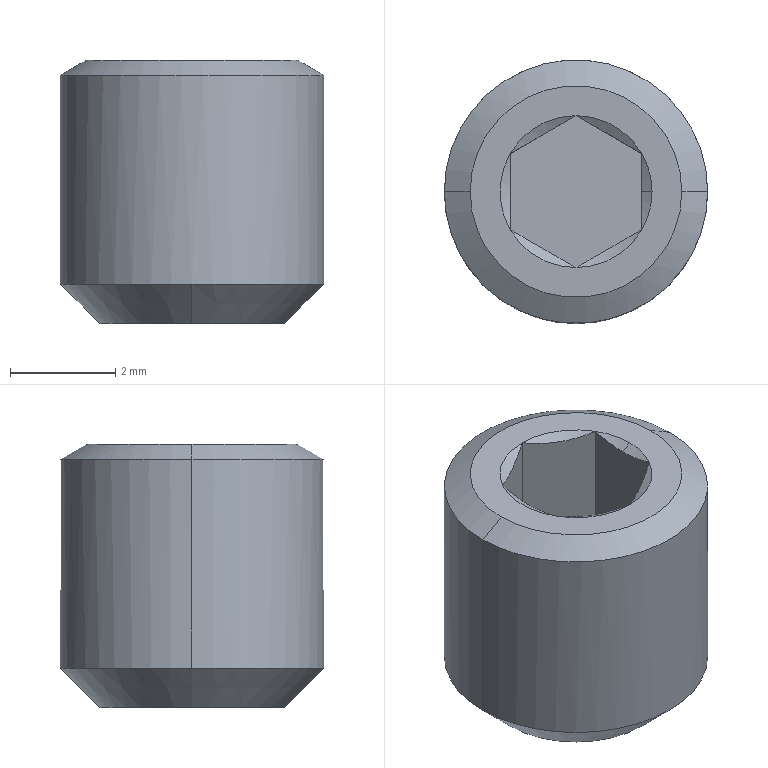Component | SolidWorks | DGC-18-280-G-PPV-A-1_HI_DIN-913 - M5x5_1-1 | 1 solid | 22 faces | box 5 x 5 x 5 mm | volume 82 mm3 | cone 11 | plane 9 | cylinder 2 | commonest cylinder face diameters 5 x2
STEP:
#1=COLOUR_RGB('',0.7922,0.8196,0.9333);
#2=FILL_AREA_STYLE_COLOUR('',#1);
#3=FILL_AREA_STYLE('',(#2));
#4=SURFACE_STYLE_FILL_AREA(#3);
#5=SURFACE_SIDE_STYLE('',(#4));
#6=SURFACE_STYLE_USAGE(.BOTH.,#5);
#7=PRESENTATION_STYLE_ASSIGNMENT((#6));
#8=CARTESIAN_POINT('',(2.476,17.604,4.802));
#9=VERTEX_POINT('',#8);
#10=CARTESIAN_POINT('',(2.673,17.604,4.802));
#11=VERTEX_POINT('',#10);
#12=CARTESIAN_POINT('',(2.575,17.604,4.802));
#13=DIRECTION('',(-0.,-0.,-1.));
#14=DIRECTION('',(-1.,0.,0.));
#15=AXIS2_PLACEMENT_3D('',#12,#13,#14);
#16=CIRCLE('',#15,0.09843);
#17=EDGE_CURVE('',#9,#11,#16,.T.);
#18=ORIENTED_EDGE('',*,*,#17,.T.);
#19=CARTESIAN_POINT('',(2.673,17.604,4.646));
#20=VERTEX_POINT('',#19);
#21=CARTESIAN_POINT('',(2.673,17.604,4.78));
#22=DIRECTION('',(-0.,-0.,-1.));
#23=VECTOR('',#22,39.37);
#24=LINE('',#21,#23);
#25=EDGE_CURVE('',#11,#20,#24,.T.);
#26=ORIENTED_EDGE('',*,*,#25,.T.);
#27=CARTESIAN_POINT('',(2.575,17.702,4.646));
#28=VERTEX_POINT('',#27);
#29=CARTESIAN_POINT('',(2.575,17.604,4.646));
#30=DIRECTION('',(0.,0.,1.));
#31=DIRECTION('',(-1.,0.,0.));
#32=AXIS2_PLACEMENT_3D('',#29,#30,#31);
#33=CIRCLE('',#32,0.09843);
#34=EDGE_CURVE('',#20,#28,#33,.T.);
#35=ORIENTED_EDGE('',*,*,#34,.T.);
#36=CARTESIAN_POINT('',(2.476,17.604,4.646));
#37=VERTEX_POINT('',#36);
#38=CARTESIAN_POINT('',(2.575,17.604,4.646));
#39=DIRECTION('',(0.,0.,1.));
#40=DIRECTION('',(-1.,0.,0.));
#41=AXIS2_PLACEMENT_3D('',#38,#39,#40);
#42=CIRCLE('',#41,0.09843);
#43=EDGE_CURVE('',#28,#37,#42,.T.);
#44=ORIENTED_EDGE('',*,*,#43,.T.);
#45=CARTESIAN_POINT('',(2.476,17.604,4.78));
#46=DIRECTION('',(-0.,-0.,-1.));
#47=VECTOR('',#46,39.37);
#48=LINE('',#45,#47);
#49=EDGE_CURVE('',#9,#37,#48,.T.);
#50=ORIENTED_EDGE('',*,*,#49,.F.);
#51=EDGE_LOOP('',(#18,#26,#35,#44,#50));
#52=FACE_OUTER_BOUND('',#51,.T.);
#53=CARTESIAN_POINT('',(2.575,17.604,4.78));
#54=DIRECTION('',(-0.,-0.,-1.));
#55=DIRECTION('',(-1.,0.,0.));
#56=AXIS2_PLACEMENT_3D('',#53,#54,#55);
#57=CYLINDRICAL_SURFACE('',#56,0.09843);
#58=ADVANCED_FACE('',(#52),#57,.T.);
#59=CARTESIAN_POINT('',(2.575,17.673,4.616));
#60=VERTEX_POINT('',#59);
#61=CARTESIAN_POINT('',(2.575,17.535,4.616));
#62=VERTEX_POINT('',#61);
#63=CARTESIAN_POINT('',(2.575,17.604,4.616));
#64=DIRECTION('',(0.,0.,1.));
#65=DIRECTION('',(0.,1.,0.));
#66=AXIS2_PLACEMENT_3D('',#63,#64,#65);
#67=CIRCLE('',#66,0.0689);
#68=EDGE_CURVE('',#60,#62,#67,.T.);
#69=ORIENTED_EDGE('',*,*,#68,.T.);
#70=CARTESIAN_POINT('',(2.575,17.505,4.646));
#71=VERTEX_POINT('',#70);
#72=CARTESIAN_POINT('',(2.575,17.505,4.646));
#73=DIRECTION('',(-0.,-0.7071,0.7071));
#74=VECTOR('',#73,39.37);
#75=LINE('',#72,#74);
#76=EDGE_CURVE('',#62,#71,#75,.T.);
#77=ORIENTED_EDGE('',*,*,#76,.T.);
#78=CARTESIAN_POINT('',(2.575,17.604,4.646));
#79=DIRECTION('',(0.,0.,1.));
#80=DIRECTION('',(-1.,0.,0.));
#81=AXIS2_PLACEMENT_3D('',#78,#79,#80);
#82=CIRCLE('',#81,0.09843);
#83=EDGE_CURVE('',#37,#71,#82,.T.);
#84=ORIENTED_EDGE('',*,*,#83,.F.);
#85=ORIENTED_EDGE('',*,*,#43,.F.);
#86=CARTESIAN_POINT('',(2.575,17.702,4.646));
#87=DIRECTION('',(0.,0.7071,0.7071));
#88=VECTOR('',#87,39.37);
#89=LINE('',#86,#88);
#90=EDGE_CURVE('',#60,#28,#89,.T.);
#91=ORIENTED_EDGE('',*,*,#90,.F.);
#92=EDGE_LOOP('',(#69,#77,#84,#85,#91));
#93=FACE_OUTER_BOUND('',#92,.T.);
#94=CARTESIAN_POINT('',(2.575,17.604,4.646));
#95=DIRECTION('',(0.,0.,1.));
#96=DIRECTION('',(0.,1.,0.));
#97=AXIS2_PLACEMENT_3D('',#94,#95,#96);
#98=CONICAL_SURFACE('',#97,0.09843,0.7854);
#99=ADVANCED_FACE('',(#93),#98,.T.);
#100=CARTESIAN_POINT('',(2.496,17.604,4.813));
#101=VERTEX_POINT('',#100);
#102=CARTESIAN_POINT('',(2.654,17.604,4.813));
#103=VERTEX_POINT('',#102);
#104=CARTESIAN_POINT('',(2.575,17.604,4.813));
#105=DIRECTION('',(-0.,-0.,-1.));
#106=DIRECTION('',(-1.,0.,0.));
#107=AXIS2_PLACEMENT_3D('',#104,#105,#106);
#108=CIRCLE('',#107,0.07911);
#109=EDGE_CURVE('',#101,#103,#108,.T.);
#110=ORIENTED_EDGE('',*,*,#109,.T.);
#111=CARTESIAN_POINT('',(2.673,17.604,4.802));
#112=DIRECTION('',(0.866,0.,-0.5));
#113=VECTOR('',#112,39.37);
#114=LINE('',#111,#113);
#115=EDGE_CURVE('',#103,#11,#114,.T.);
#116=ORIENTED_EDGE('',*,*,#115,.T.);
#117=ORIENTED_EDGE('',*,*,#17,.F.);
#118=CARTESIAN_POINT('',(2.476,17.604,4.802));
#119=DIRECTION('',(-0.866,-0.,-0.5));
#120=VECTOR('',#119,39.37);
#121=LINE('',#118,#120);
#122=EDGE_CURVE('',#101,#9,#121,.T.);
#123=ORIENTED_EDGE('',*,*,#122,.F.);
#124=EDGE_LOOP('',(#110,#116,#117,#123));
#125=FACE_OUTER_BOUND('',#124,.T.);
#126=CARTESIAN_POINT('',(2.575,17.604,4.802));
#127=DIRECTION('',(-0.,-0.,-1.));
#128=DIRECTION('',(-1.,0.,0.));
#129=AXIS2_PLACEMENT_3D('',#126,#127,#128);
#130=CONICAL_SURFACE('',#129,0.09843,1.047);
#131=ADVANCED_FACE('',(#125),#130,.T.);
#132=CARTESIAN_POINT('',(2.624,17.604,4.809));
#133=VERTEX_POINT('',#132);
#134=CARTESIAN_POINT('',(2.624,17.632,4.813));
#135=VERTEX_POINT('',#134);
#136=CARTESIAN_POINT('',(2.624,17.604,4.809));
#137=CARTESIAN_POINT('',(2.624,17.613,4.809));
#138=CARTESIAN_POINT('',(2.624,17.623,4.81));
#139=CARTESIAN_POINT('',(2.624,17.632,4.813));
#140=B_SPLINE_CURVE_WITH_KNOTS('',3,(#136,#137,#138,#139),.UNSPECIFIED.,.F.,.F.,(4,4),(0.0007302,0.001458),.UNSPECIFIED.);
#141=EDGE_CURVE('',#133,#135,#140,.T.);
#142=ORIENTED_EDGE('',*,*,#141,.F.);
#143=CARTESIAN_POINT('',(2.632,17.604,4.813));
#144=VERTEX_POINT('',#143);
#145=CARTESIAN_POINT('',(2.632,17.604,4.813));
#146=DIRECTION('',(0.866,0.,0.5));
#147=VECTOR('',#146,39.37);
#148=LINE('',#145,#147);
#149=EDGE_CURVE('',#133,#144,#148,.T.);
#150=ORIENTED_EDGE('',*,*,#149,.T.);
#151=CARTESIAN_POINT('',(2.575,17.604,4.813));
#152=DIRECTION('',(0.,0.,1.));
#153=DIRECTION('',(1.,0.,0.));
#154=AXIS2_PLACEMENT_3D('',#151,#152,#153);
#155=CIRCLE('',#154,0.05683);
#156=EDGE_CURVE('',#144,#135,#155,.T.);
#157=ORIENTED_EDGE('',*,*,#156,.T.);
#158=EDGE_LOOP('',(#142,#150,#157));
#159=FACE_OUTER_BOUND('',#158,.T.);
#160=CARTESIAN_POINT('',(2.575,17.604,4.813));
#161=DIRECTION('',(0.,0.,1.));
#162=DIRECTION('',(1.,0.,0.));
#163=AXIS2_PLACEMENT_3D('',#160,#161,#162);
#164=CONICAL_SURFACE('',#163,0.05683,1.047);
#165=ADVANCED_FACE('',(#159),#164,.F.);
#166=ORIENTED_EDGE('',*,*,#25,.F.);
#167=CARTESIAN_POINT('',(2.575,17.604,4.802));
#168=DIRECTION('',(-0.,-0.,-1.));
#169=DIRECTION('',(-1.,0.,0.));
#170=AXIS2_PLACEMENT_3D('',#167,#168,#169);
#171=CIRCLE('',#170,0.09843);
#172=EDGE_CURVE('',#11,#9,#171,.T.);
#173=ORIENTED_EDGE('',*,*,#172,.T.);
#174=ORIENTED_EDGE('',*,*,#49,.T.);
#175=ORIENTED_EDGE('',*,*,#83,.T.);
#176=CARTESIAN_POINT('',(2.575,17.604,4.646));
#177=DIRECTION('',(0.,0.,1.));
#178=DIRECTION('',(-1.,0.,0.));
#179=AXIS2_PLACEMENT_3D('',#176,#177,#178);
#180=CIRCLE('',#179,0.09843);
#181=EDGE_CURVE('',#71,#20,#180,.T.);
#182=ORIENTED_EDGE('',*,*,#181,.T.);
#183=EDGE_LOOP('',(#166,#173,#174,#175,#182));
#184=FACE_OUTER_BOUND('',#183,.T.);
#185=CARTESIAN_POINT('',(2.575,17.604,4.78));
#186=DIRECTION('',(-0.,-0.,-1.));
#187=DIRECTION('',(-1.,0.,0.));
#188=AXIS2_PLACEMENT_3D('',#185,#186,#187);
#189=CYLINDRICAL_SURFACE('',#188,0.09843);
#190=ADVANCED_FACE('',(#184),#189,.T.);
#191=ORIENTED_EDGE('',*,*,#76,.F.);
#192=CARTESIAN_POINT('',(2.575,17.604,4.616));
#193=DIRECTION('',(0.,0.,1.));
#194=DIRECTION('',(0.,1.,0.));
#195=AXIS2_PLACEMENT_3D('',#192,#193,#194);
#196=CIRCLE('',#195,0.0689);
#197=EDGE_CURVE('',#62,#60,#196,.T.);
#198=ORIENTED_EDGE('',*,*,#197,.T.);
#199=ORIENTED_EDGE('',*,*,#90,.T.);
#200=ORIENTED_EDGE('',*,*,#34,.F.);
#201=ORIENTED_EDGE('',*,*,#181,.F.);
#202=EDGE_LOOP('',(#191,#198,#199,#200,#201));
#203=FACE_OUTER_BOUND('',#202,.T.);
#204=CARTESIAN_POINT('',(2.575,17.604,4.646));
#205=DIRECTION('',(0.,0.,1.));
#206=DIRECTION('',(0.,1.,0.));
#207=AXIS2_PLACEMENT_3D('',#204,#205,#206);
#208=CONICAL_SURFACE('',#207,0.09843,0.7854);
#209=ADVANCED_FACE('',(#203),#208,.T.);
#210=ORIENTED_EDGE('',*,*,#115,.F.);
#211=CARTESIAN_POINT('',(2.575,17.604,4.813));
#212=DIRECTION('',(-0.,-0.,-1.));
#213=DIRECTION('',(-1.,0.,0.));
#214=AXIS2_PLACEMENT_3D('',#211,#212,#213);
#215=CIRCLE('',#214,0.07911);
#216=EDGE_CURVE('',#103,#101,#215,.T.);
#217=ORIENTED_EDGE('',*,*,#216,.T.);
#218=ORIENTED_EDGE('',*,*,#122,.T.);
#219=ORIENTED_EDGE('',*,*,#172,.F.);
#220=EDGE_LOOP('',(#210,#217,#218,#219));
#221=FACE_OUTER_BOUND('',#220,.T.);
#222=CARTESIAN_POINT('',(2.575,17.604,4.802));
#223=DIRECTION('',(-0.,-0.,-1.));
#224=DIRECTION('',(-1.,0.,0.));
#225=AXIS2_PLACEMENT_3D('',#222,#223,#224);
#226=CONICAL_SURFACE('',#225,0.09843,1.047);
#227=ADVANCED_FACE('',(#221),#226,.T.);
#228=ORIENTED_EDGE('',*,*,#68,.F.);
#229=ORIENTED_EDGE('',*,*,#197,.F.);
#230=EDGE_LOOP('',(#228,#229));
#231=FACE_OUTER_BOUND('',#230,.T.);
#232=CARTESIAN_POINT('',(2.575,17.604,4.616));
#233=DIRECTION('',(0.,0.,1.));
#234=DIRECTION('',(1.,0.,-0.));
#235=AXIS2_PLACEMENT_3D('',#232,#233,#234);
#236=PLANE('',#235);
#237=ADVANCED_FACE('',(#231),#236,.F.);
#238=ORIENTED_EDGE('',*,*,#109,.F.);
#239=ORIENTED_EDGE('',*,*,#216,.F.);
#240=EDGE_LOOP('',(#238,#239));
#241=FACE_OUTER_BOUND('',#240,.T.);
#242=CARTESIAN_POINT('',(2.575,17.547,4.813));
#243=VERTEX_POINT('',#242);
#244=CARTESIAN_POINT('',(2.624,17.575,4.813));
#245=VERTEX_POINT('',#244);
#246=CARTESIAN_POINT('',(2.575,17.604,4.813));
#247=DIRECTION('',(0.,0.,1.));
#248=DIRECTION('',(1.,0.,0.));
#249=AXIS2_PLACEMENT_3D('',#246,#247,#248);
#250=CIRCLE('',#249,0.05683);
#251=EDGE_CURVE('',#243,#245,#250,.T.);
#252=ORIENTED_EDGE('',*,*,#251,.F.);
#253=CARTESIAN_POINT('',(2.526,17.575,4.813));
#254=VERTEX_POINT('',#253);
#255=CARTESIAN_POINT('',(2.575,17.604,4.813));
#256=DIRECTION('',(0.,0.,1.));
#257=DIRECTION('',(1.,0.,0.));
#258=AXIS2_PLACEMENT_3D('',#255,#256,#257);
#259=CIRCLE('',#258,0.05683);
#260=EDGE_CURVE('',#254,#243,#259,.T.);
#261=ORIENTED_EDGE('',*,*,#260,.F.);
#262=CARTESIAN_POINT('',(2.526,17.632,4.813));
#263=VERTEX_POINT('',#262);
#264=CARTESIAN_POINT('',(2.575,17.604,4.813));
#265=DIRECTION('',(0.,0.,1.));
#266=DIRECTION('',(1.,0.,0.));
#267=AXIS2_PLACEMENT_3D('',#264,#265,#266);
#268=CIRCLE('',#267,0.05683);
#269=EDGE_CURVE('',#263,#254,#268,.T.);
#270=ORIENTED_EDGE('',*,*,#269,.F.);
#271=CARTESIAN_POINT('',(2.575,17.661,4.813));
#272=VERTEX_POINT('',#271);
#273=CARTESIAN_POINT('',(2.575,17.604,4.813));
#274=DIRECTION('',(0.,0.,1.));
#275=DIRECTION('',(1.,0.,0.));
#276=AXIS2_PLACEMENT_3D('',#273,#274,#275);
#277=CIRCLE('',#276,0.05683);
#278=EDGE_CURVE('',#272,#263,#277,.T.);
#279=ORIENTED_EDGE('',*,*,#278,.F.);
#280=CARTESIAN_POINT('',(2.575,17.604,4.813));
#281=DIRECTION('',(0.,0.,1.));
#282=DIRECTION('',(1.,0.,0.));
#283=AXIS2_PLACEMENT_3D('',#280,#281,#282);
#284=CIRCLE('',#283,0.05683);
#285=EDGE_CURVE('',#135,#272,#284,.T.);
#286=ORIENTED_EDGE('',*,*,#285,.F.);
#287=ORIENTED_EDGE('',*,*,#156,.F.);
#288=CARTESIAN_POINT('',(2.575,17.604,4.813));
#289=DIRECTION('',(0.,0.,1.));
#290=DIRECTION('',(1.,0.,0.));
#291=AXIS2_PLACEMENT_3D('',#288,#289,#290);
#292=CIRCLE('',#291,0.05683);
#293=EDGE_CURVE('',#245,#144,#292,.T.);
#294=ORIENTED_EDGE('',*,*,#293,.F.);
#295=EDGE_LOOP('',(#252,#261,#270,#279,#286,#287,#294));
#296=FACE_BOUND('',#295,.T.);
#297=CARTESIAN_POINT('',(2.654,17.604,4.813));
#298=DIRECTION('',(-0.,-0.,-1.));
#299=DIRECTION('',(-1.,-0.,0.));
#300=AXIS2_PLACEMENT_3D('',#297,#298,#299);
#301=PLANE('',#300);
#302=ADVANCED_FACE('',(#241,#296),#301,.F.);
#303=ORIENTED_EDGE('',*,*,#149,.F.);
#304=CARTESIAN_POINT('',(2.624,17.575,4.813));
#305=CARTESIAN_POINT('',(2.624,17.585,4.81));
#306=CARTESIAN_POINT('',(2.624,17.594,4.809));
#307=CARTESIAN_POINT('',(2.624,17.604,4.809));
#308=B_SPLINE_CURVE_WITH_KNOTS('',3,(#304,#305,#306,#307),.UNSPECIFIED.,.F.,.F.,(4,4),(0.,0.0007302),.UNSPECIFIED.);
#309=EDGE_CURVE('',#245,#133,#308,.T.);
#310=ORIENTED_EDGE('',*,*,#309,.F.);
#311=ORIENTED_EDGE('',*,*,#293,.T.);
#312=EDGE_LOOP('',(#303,#310,#311));
#313=FACE_OUTER_BOUND('',#312,.T.);
#314=CARTESIAN_POINT('',(2.575,17.604,4.813));
#315=DIRECTION('',(0.,0.,1.));
#316=DIRECTION('',(1.,0.,0.));
#317=AXIS2_PLACEMENT_3D('',#314,#315,#316);
#318=CONICAL_SURFACE('',#317,0.05683,1.047);
#319=ADVANCED_FACE('',(#313),#318,.F.);
#320=ORIENTED_EDGE('',*,*,#251,.T.);
#321=CARTESIAN_POINT('',(2.575,17.547,4.813));
#322=CARTESIAN_POINT('',(2.583,17.552,4.81));
#323=CARTESIAN_POINT('',(2.591,17.556,4.809));
#324=CARTESIAN_POINT('',(2.608,17.566,4.809));
#325=CARTESIAN_POINT('',(2.616,17.571,4.81));
#326=CARTESIAN_POINT('',(2.624,17.575,4.813));
#327=B_SPLINE_CURVE_WITH_KNOTS('',3,(#321,#322,#323,#324,#325,#326),.UNSPECIFIED.,.F.,.F.,(4,2,4),(0.,0.0007289,0.001458),.UNSPECIFIED.);
#328=EDGE_CURVE('',#243,#245,#327,.T.);
#329=ORIENTED_EDGE('',*,*,#328,.F.);
#330=EDGE_LOOP('',(#320,#329));
#331=FACE_OUTER_BOUND('',#330,.T.);
#332=CARTESIAN_POINT('',(2.575,17.604,4.813));
#333=DIRECTION('',(0.,0.,1.));
#334=DIRECTION('',(1.,0.,0.));
#335=AXIS2_PLACEMENT_3D('',#332,#333,#334);
#336=CONICAL_SURFACE('',#335,0.05683,1.047);
#337=ADVANCED_FACE('',(#331),#336,.F.);
#338=ORIENTED_EDGE('',*,*,#260,.T.);
#339=CARTESIAN_POINT('',(2.526,17.575,4.813));
#340=CARTESIAN_POINT('',(2.534,17.571,4.81));
#341=CARTESIAN_POINT('',(2.542,17.566,4.809));
#342=CARTESIAN_POINT('',(2.558,17.556,4.809));
#343=CARTESIAN_POINT('',(2.567,17.552,4.81));
#344=CARTESIAN_POINT('',(2.575,17.547,4.813));
#345=B_SPLINE_CURVE_WITH_KNOTS('',3,(#339,#340,#341,#342,#343,#344),.UNSPECIFIED.,.F.,.F.,(4,2,4),(0.,0.0007289,0.001458),.UNSPECIFIED.);
#346=EDGE_CURVE('',#254,#243,#345,.T.);
#347=ORIENTED_EDGE('',*,*,#346,.F.);
#348=EDGE_LOOP('',(#338,#347));
#349=FACE_OUTER_BOUND('',#348,.T.);
#350=CARTESIAN_POINT('',(2.575,17.604,4.813));
#351=DIRECTION('',(0.,0.,1.));
#352=DIRECTION('',(1.,0.,0.));
#353=AXIS2_PLACEMENT_3D('',#350,#351,#352);
#354=CONICAL_SURFACE('',#353,0.05683,1.047);
#355=ADVANCED_FACE('',(#349),#354,.F.);
#356=ORIENTED_EDGE('',*,*,#269,.T.);
#357=CARTESIAN_POINT('',(2.526,17.632,4.813));
#358=CARTESIAN_POINT('',(2.526,17.623,4.81));
#359=CARTESIAN_POINT('',(2.526,17.614,4.809));
#360=CARTESIAN_POINT('',(2.526,17.594,4.809));
#361=CARTESIAN_POINT('',(2.526,17.585,4.81));
#362=CARTESIAN_POINT('',(2.526,17.575,4.813));
#363=B_SPLINE_CURVE_WITH_KNOTS('',3,(#357,#358,#359,#360,#361,#362),.UNSPECIFIED.,.F.,.F.,(4,2,4),(0.,0.0007289,0.001458),.UNSPECIFIED.);
#364=EDGE_CURVE('',#263,#254,#363,.T.);
#365=ORIENTED_EDGE('',*,*,#364,.F.);
#366=EDGE_LOOP('',(#356,#365));
#367=FACE_OUTER_BOUND('',#366,.T.);
#368=CARTESIAN_POINT('',(2.575,17.604,4.813));
#369=DIRECTION('',(0.,0.,1.));
#370=DIRECTION('',(1.,0.,0.));
#371=AXIS2_PLACEMENT_3D('',#368,#369,#370);
#372=CONICAL_SURFACE('',#371,0.05683,1.047);
#373=ADVANCED_FACE('',(#367),#372,.F.);
#374=ORIENTED_EDGE('',*,*,#278,.T.);
#375=CARTESIAN_POINT('',(2.575,17.661,4.813));
#376=CARTESIAN_POINT('',(2.567,17.656,4.81));
#377=CARTESIAN_POINT('',(2.559,17.651,4.809));
#378=CARTESIAN_POINT('',(2.542,17.642,4.809));
#379=CARTESIAN_POINT('',(2.534,17.637,4.81));
#380=CARTESIAN_POINT('',(2.526,17.632,4.813));
#381=B_SPLINE_CURVE_WITH_KNOTS('',3,(#375,#376,#377,#378,#379,#380),.UNSPECIFIED.,.F.,.F.,(4,2,4),(0.,0.0007289,0.001458),.UNSPECIFIED.);
#382=EDGE_CURVE('',#272,#263,#381,.T.);
#383=ORIENTED_EDGE('',*,*,#382,.F.);
#384=EDGE_LOOP('',(#374,#383));
#385=FACE_OUTER_BOUND('',#384,.T.);
#386=CARTESIAN_POINT('',(2.575,17.604,4.813));
#387=DIRECTION('',(0.,0.,1.));
#388=DIRECTION('',(1.,0.,0.));
#389=AXIS2_PLACEMENT_3D('',#386,#387,#388);
#390=CONICAL_SURFACE('',#389,0.05683,1.047);
#391=ADVANCED_FACE('',(#385),#390,.F.);
#392=ORIENTED_EDGE('',*,*,#285,.T.);
#393=CARTESIAN_POINT('',(2.624,17.632,4.813));
#394=CARTESIAN_POINT('',(2.616,17.637,4.81));
#395=CARTESIAN_POINT('',(2.608,17.642,4.809));
#396=CARTESIAN_POINT('',(2.591,17.651,4.809));
#397=CARTESIAN_POINT('',(2.583,17.656,4.81));
#398=CARTESIAN_POINT('',(2.575,17.661,4.813));
#399=B_SPLINE_CURVE_WITH_KNOTS('',3,(#393,#394,#395,#396,#397,#398),.UNSPECIFIED.,.F.,.F.,(4,2,4),(0.,0.0007289,0.001458),.UNSPECIFIED.);
#400=EDGE_CURVE('',#135,#272,#399,.T.);
#401=ORIENTED_EDGE('',*,*,#400,.F.);
#402=EDGE_LOOP('',(#392,#401));
#403=FACE_OUTER_BOUND('',#402,.T.);
#404=CARTESIAN_POINT('',(2.575,17.604,4.813));
#405=DIRECTION('',(0.,0.,1.));
#406=DIRECTION('',(1.,0.,0.));
#407=AXIS2_PLACEMENT_3D('',#404,#405,#406);
#408=CONICAL_SURFACE('',#407,0.05683,1.047);
#409=ADVANCED_FACE('',(#403),#408,.F.);
#410=CARTESIAN_POINT('',(2.624,17.632,4.734));
#411=VERTEX_POINT('',#410);
#412=CARTESIAN_POINT('',(2.624,17.575,4.734));
#413=VERTEX_POINT('',#412);
#414=CARTESIAN_POINT('',(2.624,17.632,4.734));
#415=DIRECTION('',(0.,-1.,0.));
#416=VECTOR('',#415,39.37);
#417=LINE('',#414,#416);
#418=EDGE_CURVE('',#411,#413,#417,.T.);
#419=ORIENTED_EDGE('',*,*,#418,.T.);
#420=CARTESIAN_POINT('',(2.624,17.575,4.734));
#421=DIRECTION('',(0.,0.,1.));
#422=VECTOR('',#421,39.37);
#423=LINE('',#420,#422);
#424=EDGE_CURVE('',#413,#245,#423,.T.);
#425=ORIENTED_EDGE('',*,*,#424,.T.);
#426=ORIENTED_EDGE('',*,*,#309,.T.);
#427=ORIENTED_EDGE('',*,*,#141,.T.);
#428=CARTESIAN_POINT('',(2.624,17.632,4.734));
#429=DIRECTION('',(-0.,0.,-1.));
#430=VECTOR('',#429,39.37);
#431=LINE('',#428,#430);
#432=EDGE_CURVE('',#135,#411,#431,.T.);
#433=ORIENTED_EDGE('',*,*,#432,.T.);
#434=EDGE_LOOP('',(#419,#425,#426,#427,#433));
#435=FACE_OUTER_BOUND('',#434,.T.);
#436=CARTESIAN_POINT('',(2.624,17.632,4.734));
#437=DIRECTION('',(-1.,-0.,0.));
#438=DIRECTION('',(-0.,1.,0.));
#439=AXIS2_PLACEMENT_3D('',#436,#437,#438);
#440=PLANE('',#439);
#441=ADVANCED_FACE('',(#435),#440,.T.);
#442=CARTESIAN_POINT('',(2.575,17.547,4.734));
#443=VERTEX_POINT('',#442);
#444=CARTESIAN_POINT('',(2.624,17.575,4.734));
#445=DIRECTION('',(-0.866,-0.5,0.));
#446=VECTOR('',#445,39.37);
#447=LINE('',#444,#446);
#448=EDGE_CURVE('',#413,#443,#447,.T.);
#449=ORIENTED_EDGE('',*,*,#448,.T.);
#450=CARTESIAN_POINT('',(2.575,17.547,4.734));
#451=DIRECTION('',(0.,0.,1.));
#452=VECTOR('',#451,39.37);
#453=LINE('',#450,#452);
#454=EDGE_CURVE('',#443,#243,#453,.T.);
#455=ORIENTED_EDGE('',*,*,#454,.T.);
#456=ORIENTED_EDGE('',*,*,#328,.T.);
#457=ORIENTED_EDGE('',*,*,#424,.F.);
#458=EDGE_LOOP('',(#449,#455,#456,#457));
#459=FACE_OUTER_BOUND('',#458,.T.);
#460=CARTESIAN_POINT('',(2.624,17.575,4.734));
#461=DIRECTION('',(-0.5,0.866,0.));
#462=DIRECTION('',(0.866,0.5,-0.));
#463=AXIS2_PLACEMENT_3D('',#460,#461,#462);
#464=PLANE('',#463);
#465=ADVANCED_FACE('',(#459),#464,.T.);
#466=CARTESIAN_POINT('',(2.526,17.575,4.734));
#467=VERTEX_POINT('',#466);
#468=CARTESIAN_POINT('',(2.526,17.632,4.734));
#469=VERTEX_POINT('',#468);
#470=CARTESIAN_POINT('',(2.526,17.575,4.734));
#471=DIRECTION('',(-0.,1.,0.));
#472=VECTOR('',#471,39.37);
#473=LINE('',#470,#472);
#474=EDGE_CURVE('',#467,#469,#473,.T.);
#475=ORIENTED_EDGE('',*,*,#474,.F.);
#476=CARTESIAN_POINT('',(2.575,17.547,4.734));
#477=DIRECTION('',(-0.866,0.5,0.));
#478=VECTOR('',#477,39.37);
#479=LINE('',#476,#478);
#480=EDGE_CURVE('',#443,#467,#479,.T.);
#481=ORIENTED_EDGE('',*,*,#480,.F.);
#482=ORIENTED_EDGE('',*,*,#448,.F.);
#483=ORIENTED_EDGE('',*,*,#418,.F.);
#484=CARTESIAN_POINT('',(2.575,17.661,4.734));
#485=VERTEX_POINT('',#484);
#486=CARTESIAN_POINT('',(2.575,17.661,4.734));
#487=DIRECTION('',(0.866,-0.5,-0.));
#488=VECTOR('',#487,39.37);
#489=LINE('',#486,#488);
#490=EDGE_CURVE('',#485,#411,#489,.T.);
#491=ORIENTED_EDGE('',*,*,#490,.F.);
#492=CARTESIAN_POINT('',(2.526,17.632,4.734));
#493=DIRECTION('',(0.866,0.5,-0.));
#494=VECTOR('',#493,39.37);
#495=LINE('',#492,#494);
#496=EDGE_CURVE('',#469,#485,#495,.T.);
#497=ORIENTED_EDGE('',*,*,#496,.F.);
#498=EDGE_LOOP('',(#475,#481,#482,#483,#491,#497));
#499=FACE_OUTER_BOUND('',#498,.T.);
#500=CARTESIAN_POINT('',(2.575,17.604,4.734));
#501=DIRECTION('',(-0.,-0.,-1.));
#502=DIRECTION('',(0.,-1.,0.));
#503=AXIS2_PLACEMENT_3D('',#500,#501,#502);
#504=PLANE('',#503);
#505=ADVANCED_FACE('',(#499),#504,.F.);
#506=ORIENTED_EDGE('',*,*,#490,.T.);
#507=ORIENTED_EDGE('',*,*,#432,.F.);
#508=ORIENTED_EDGE('',*,*,#400,.T.);
#509=CARTESIAN_POINT('',(2.575,17.661,4.734));
#510=DIRECTION('',(-0.,0.,-1.));
#511=VECTOR('',#510,39.37);
#512=LINE('',#509,#511);
#513=EDGE_CURVE('',#272,#485,#512,.T.);
#514=ORIENTED_EDGE('',*,*,#513,.T.);
#515=EDGE_LOOP('',(#506,#507,#508,#514));
#516=FACE_OUTER_BOUND('',#515,.T.);
#517=CARTESIAN_POINT('',(2.575,17.661,4.734));
#518=DIRECTION('',(-0.5,-0.866,0.));
#519=DIRECTION('',(-0.866,0.5,0.));
#520=AXIS2_PLACEMENT_3D('',#517,#518,#519);
#521=PLANE('',#520);
#522=ADVANCED_FACE('',(#516),#521,.T.);
#523=ORIENTED_EDGE('',*,*,#480,.T.);
#524=CARTESIAN_POINT('',(2.526,17.575,4.734));
#525=DIRECTION('',(0.,0.,1.));
#526=VECTOR('',#525,39.37);
#527=LINE('',#524,#526);
#528=EDGE_CURVE('',#467,#254,#527,.T.);
#529=ORIENTED_EDGE('',*,*,#528,.T.);
#530=ORIENTED_EDGE('',*,*,#346,.T.);
#531=ORIENTED_EDGE('',*,*,#454,.F.);
#532=EDGE_LOOP('',(#523,#529,#530,#531));
#533=FACE_OUTER_BOUND('',#532,.T.);
#534=CARTESIAN_POINT('',(2.575,17.547,4.734));
#535=DIRECTION('',(0.5,0.866,-0.));
#536=DIRECTION('',(0.866,-0.5,-0.));
#537=AXIS2_PLACEMENT_3D('',#534,#535,#536);
#538=PLANE('',#537);
#539=ADVANCED_FACE('',(#533),#538,.T.);
#540=ORIENTED_EDGE('',*,*,#496,.T.);
#541=ORIENTED_EDGE('',*,*,#513,.F.);
#542=ORIENTED_EDGE('',*,*,#382,.T.);
#543=CARTESIAN_POINT('',(2.526,17.632,4.734));
#544=DIRECTION('',(-0.,0.,-1.));
#545=VECTOR('',#544,39.37);
#546=LINE('',#543,#545);
#547=EDGE_CURVE('',#263,#469,#546,.T.);
#548=ORIENTED_EDGE('',*,*,#547,.T.);
#549=EDGE_LOOP('',(#540,#541,#542,#548));
#550=FACE_OUTER_BOUND('',#549,.T.);
#551=CARTESIAN_POINT('',(2.526,17.632,4.734));
#552=DIRECTION('',(0.5,-0.866,-0.));
#553=DIRECTION('',(-0.866,-0.5,0.));
#554=AXIS2_PLACEMENT_3D('',#551,#552,#553);
#555=PLANE('',#554);
#556=ADVANCED_FACE('',(#550),#555,.T.);
#557=ORIENTED_EDGE('',*,*,#474,.T.);
#558=ORIENTED_EDGE('',*,*,#547,.F.);
#559=ORIENTED_EDGE('',*,*,#364,.T.);
#560=ORIENTED_EDGE('',*,*,#528,.F.);
#561=EDGE_LOOP('',(#557,#558,#559,#560));
#562=FACE_OUTER_BOUND('',#561,.T.);
#563=CARTESIAN_POINT('',(2.526,17.575,4.734));
#564=DIRECTION('',(1.,0.,-0.));
#565=DIRECTION('',(0.,-1.,0.));
#566=AXIS2_PLACEMENT_3D('',#563,#564,#565);
#567=PLANE('',#566);
#568=ADVANCED_FACE('',(#562),#567,.T.);
#569=CLOSED_SHELL('',(#58,#99,#131,#165,#190,#209,#227,#237,#302,#319,#337,#355,#373,#391,#409,#441,#465,#505,#522,#539,#556,#568));
#570=MANIFOLD_SOLID_BREP('',#569);
#571=STYLED_ITEM('',(#7),#570);
#572=PRESENTATION_LAYER_ASSIGNMENT('','',(#571));
#573=(LENGTH_UNIT()NAMED_UNIT(*)SI_UNIT($,.METRE.));
#574=LENGTH_MEASURE_WITH_UNIT(LENGTH_MEASURE(0.0254),#573);
#575=DIMENSIONAL_EXPONENTS(1.,0.,0.,0.,0.,0.,0.);
#576=(CONVERSION_BASED_UNIT('',#574)LENGTH_UNIT()NAMED_UNIT(#575));
#577=UNCERTAINTY_MEASURE_WITH_UNIT(LENGTH_MEASURE(0.00001),#576,'','');
#578=(NAMED_UNIT(*)PLANE_ANGLE_UNIT()SI_UNIT($,.RADIAN.));
#579=(NAMED_UNIT(*)SI_UNIT($,.STERADIAN.)SOLID_ANGLE_UNIT());
#580=(GEOMETRIC_REPRESENTATION_CONTEXT(3)GLOBAL_UNCERTAINTY_ASSIGNED_CONTEXT((#577))GLOBAL_UNIT_ASSIGNED_CONTEXT((#576,#578,#579))REPRESENTATION_CONTEXT('',''));
#581=MECHANICAL_DESIGN_GEOMETRIC_PRESENTATION_REPRESENTATION('',(#571),#580);
#582=CARTESIAN_POINT('',(0.,0.,0.));
#583=DIRECTION('',(0.,0.,1.));
#584=DIRECTION('',(1.,0.,0.));
#585=AXIS2_PLACEMENT_3D('',#582,#583,#584);
#586=(LENGTH_UNIT()NAMED_UNIT(*)SI_UNIT($,.METRE.));
#587=LENGTH_MEASURE_WITH_UNIT(LENGTH_MEASURE(0.0254),#586);
#588=DIMENSIONAL_EXPONENTS(1.,0.,0.,0.,0.,0.,0.);
#589=(CONVERSION_BASED_UNIT('',#587)LENGTH_UNIT()NAMED_UNIT(#588));
#590=UNCERTAINTY_MEASURE_WITH_UNIT(LENGTH_MEASURE(0.00001),#589,'','');
#591=(NAMED_UNIT(*)PLANE_ANGLE_UNIT()SI_UNIT($,.RADIAN.));
#592=(NAMED_UNIT(*)SI_UNIT($,.STERADIAN.)SOLID_ANGLE_UNIT());
#593=(GEOMETRIC_REPRESENTATION_CONTEXT(3)GLOBAL_UNCERTAINTY_ASSIGNED_CONTEXT((#590))GLOBAL_UNIT_ASSIGNED_CONTEXT((#589,#591,#592))REPRESENTATION_CONTEXT('',''));
#594=ADVANCED_BREP_SHAPE_REPRESENTATION('',(#570,#585),#593);